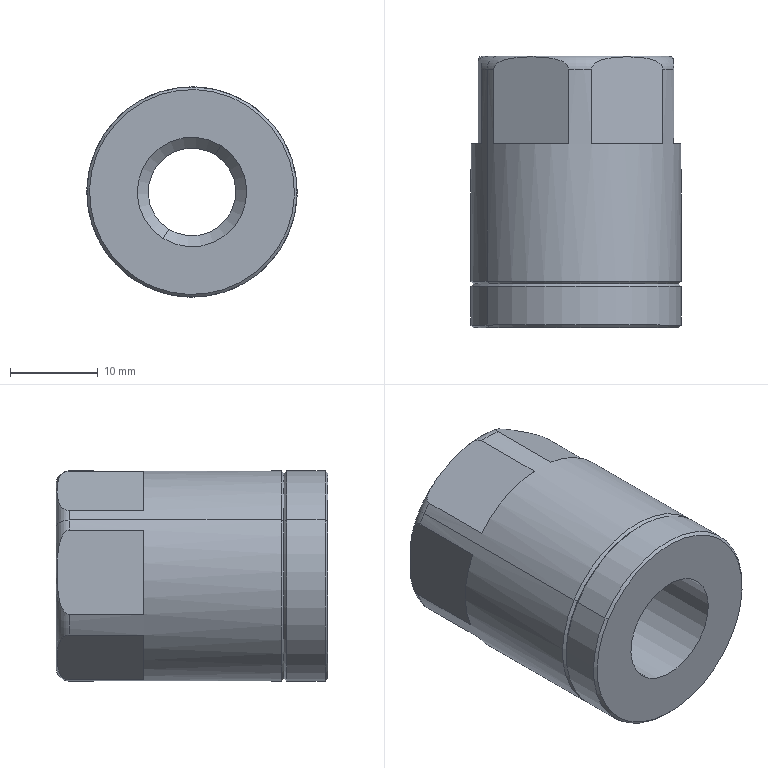Component | SolidWorks | MACJ25x25-10S-Rod-1_25MACJ2510A-Nut-1 | 1 solid | 34 faces | volume 10407 mm3 | plane 14 | cone 10 | cylinder 8 | torus 2 | commonest cylinder face diameters 24 x4 10 x2 12.5 x2